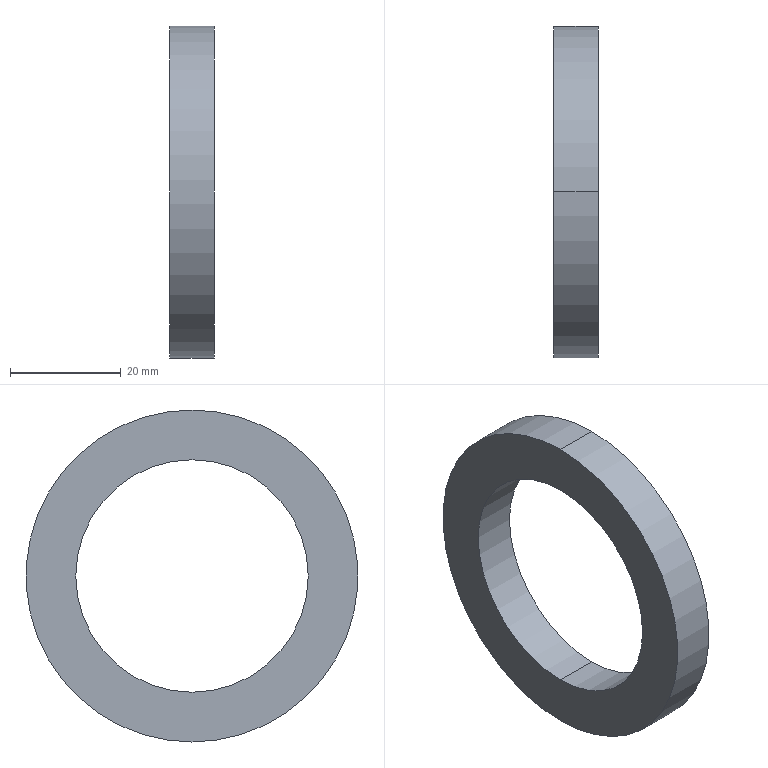Component | SolidWorks | 5ThrustWasher-1 | 1 solid | 6 faces | box 8 x 60 x 60 mm | volume 11536 mm3 | cylinder 4 | plane 2 | commonest cylinder face diameters 42 x2 60 x2
build123d program:
from build123d import *

# Parameters (mm, degrees)
SKETCH1_R           = 30
SKETCH1_R_2         = 21
BOSS_EXTRUDE1_DEPTH = 8


with BuildPart() as part:
    # Sketch1 → Boss-Extrude1 (new body)
    with BuildSketch(Plane(origin=(0, 0, 0), x_dir=(0, 0, -1), z_dir=(1, 0, 0))):
        Circle(SKETCH1_R)
        Circle(SKETCH1_R_2, mode=Mode.SUBTRACT)
    extrude(amount=BOSS_EXTRUDE1_DEPTH)


solid = part.part

# Placed as in the assembly
solid = solid.moved(Location((87.957, 1.776, 250), (0, 0, 0)))
STEP:
#1=COLOUR_RGB('',0.7922,0.8196,0.9333);
#2=FILL_AREA_STYLE_COLOUR('',#1);
#3=FILL_AREA_STYLE('',(#2));
#4=SURFACE_STYLE_FILL_AREA(#3);
#5=SURFACE_SIDE_STYLE('',(#4));
#6=SURFACE_STYLE_USAGE(.BOTH.,#5);
#7=PRESENTATION_STYLE_ASSIGNMENT((#6));
#8=CARTESIAN_POINT('',(3.778,0.06992,10.669));
#9=VERTEX_POINT('',#8);
#10=CARTESIAN_POINT('',(3.778,0.06992,9.016));
#11=VERTEX_POINT('',#10);
#12=CARTESIAN_POINT('',(3.778,0.06992,9.843));
#13=DIRECTION('',(1.,0.,0.));
#14=DIRECTION('',(0.,0.,-1.));
#15=AXIS2_PLACEMENT_3D('',#12,#13,#14);
#16=CIRCLE('',#15,0.8268);
#17=EDGE_CURVE('',#9,#11,#16,.T.);
#18=ORIENTED_EDGE('',*,*,#17,.T.);
#19=CARTESIAN_POINT('',(3.463,0.06992,9.016));
#20=VERTEX_POINT('',#19);
#21=CARTESIAN_POINT('',(3.778,0.06992,9.016));
#22=DIRECTION('',(-1.,0.,0.));
#23=VECTOR('',#22,39.37);
#24=LINE('',#21,#23);
#25=EDGE_CURVE('',#11,#20,#24,.T.);
#26=ORIENTED_EDGE('',*,*,#25,.T.);
#27=CARTESIAN_POINT('',(3.463,0.06992,10.669));
#28=VERTEX_POINT('',#27);
#29=CARTESIAN_POINT('',(3.463,0.06992,9.843));
#30=DIRECTION('',(1.,0.,0.));
#31=DIRECTION('',(0.,0.,-1.));
#32=AXIS2_PLACEMENT_3D('',#29,#30,#31);
#33=CIRCLE('',#32,0.8268);
#34=EDGE_CURVE('',#28,#20,#33,.T.);
#35=ORIENTED_EDGE('',*,*,#34,.F.);
#36=CARTESIAN_POINT('',(3.778,0.06992,10.669));
#37=DIRECTION('',(-1.,0.,0.));
#38=VECTOR('',#37,39.37);
#39=LINE('',#36,#38);
#40=EDGE_CURVE('',#9,#28,#39,.T.);
#41=ORIENTED_EDGE('',*,*,#40,.F.);
#42=EDGE_LOOP('',(#18,#26,#35,#41));
#43=FACE_OUTER_BOUND('',#42,.T.);
#44=CARTESIAN_POINT('',(3.778,0.06992,9.843));
#45=DIRECTION('',(-1.,0.,0.));
#46=DIRECTION('',(0.,0.,1.));
#47=AXIS2_PLACEMENT_3D('',#44,#45,#46);
#48=CYLINDRICAL_SURFACE('',#47,0.8268);
#49=ADVANCED_FACE('',(#43),#48,.F.);
#50=CARTESIAN_POINT('',(3.778,0.06992,8.661));
#51=VERTEX_POINT('',#50);
#52=CARTESIAN_POINT('',(3.778,0.06992,11.024));
#53=VERTEX_POINT('',#52);
#54=CARTESIAN_POINT('',(3.778,0.06992,9.843));
#55=DIRECTION('',(1.,0.,0.));
#56=DIRECTION('',(0.,0.,-1.));
#57=AXIS2_PLACEMENT_3D('',#54,#55,#56);
#58=CIRCLE('',#57,1.181);
#59=EDGE_CURVE('',#51,#53,#58,.T.);
#60=ORIENTED_EDGE('',*,*,#59,.F.);
#61=CARTESIAN_POINT('',(3.463,0.06992,8.661));
#62=VERTEX_POINT('',#61);
#63=CARTESIAN_POINT('',(3.778,0.06992,8.661));
#64=DIRECTION('',(-1.,0.,0.));
#65=VECTOR('',#64,39.37);
#66=LINE('',#63,#65);
#67=EDGE_CURVE('',#51,#62,#66,.T.);
#68=ORIENTED_EDGE('',*,*,#67,.T.);
#69=CARTESIAN_POINT('',(3.463,0.06992,11.024));
#70=VERTEX_POINT('',#69);
#71=CARTESIAN_POINT('',(3.463,0.06992,9.843));
#72=DIRECTION('',(1.,0.,0.));
#73=DIRECTION('',(0.,0.,-1.));
#74=AXIS2_PLACEMENT_3D('',#71,#72,#73);
#75=CIRCLE('',#74,1.181);
#76=EDGE_CURVE('',#62,#70,#75,.T.);
#77=ORIENTED_EDGE('',*,*,#76,.T.);
#78=CARTESIAN_POINT('',(3.778,0.06992,11.024));
#79=DIRECTION('',(-1.,0.,0.));
#80=VECTOR('',#79,39.37);
#81=LINE('',#78,#80);
#82=EDGE_CURVE('',#53,#70,#81,.T.);
#83=ORIENTED_EDGE('',*,*,#82,.F.);
#84=EDGE_LOOP('',(#60,#68,#77,#83));
#85=FACE_OUTER_BOUND('',#84,.T.);
#86=CARTESIAN_POINT('',(3.778,0.06992,9.843));
#87=DIRECTION('',(-1.,0.,0.));
#88=DIRECTION('',(0.,0.,1.));
#89=AXIS2_PLACEMENT_3D('',#86,#87,#88);
#90=CYLINDRICAL_SURFACE('',#89,1.181);
#91=ADVANCED_FACE('',(#85),#90,.T.);
#92=CARTESIAN_POINT('',(3.778,0.06992,9.843));
#93=DIRECTION('',(1.,0.,0.));
#94=DIRECTION('',(0.,0.,-1.));
#95=AXIS2_PLACEMENT_3D('',#92,#93,#94);
#96=CIRCLE('',#95,1.181);
#97=EDGE_CURVE('',#53,#51,#96,.T.);
#98=ORIENTED_EDGE('',*,*,#97,.T.);
#99=ORIENTED_EDGE('',*,*,#59,.T.);
#100=EDGE_LOOP('',(#98,#99));
#101=FACE_OUTER_BOUND('',#100,.T.);
#102=ORIENTED_EDGE('',*,*,#17,.F.);
#103=CARTESIAN_POINT('',(3.778,0.06992,9.843));
#104=DIRECTION('',(1.,0.,0.));
#105=DIRECTION('',(0.,0.,-1.));
#106=AXIS2_PLACEMENT_3D('',#103,#104,#105);
#107=CIRCLE('',#106,0.8268);
#108=EDGE_CURVE('',#11,#9,#107,.T.);
#109=ORIENTED_EDGE('',*,*,#108,.F.);
#110=EDGE_LOOP('',(#102,#109));
#111=FACE_BOUND('',#110,.T.);
#112=CARTESIAN_POINT('',(3.778,0.06992,9.843));
#113=DIRECTION('',(1.,0.,0.));
#114=DIRECTION('',(0.,0.,-1.));
#115=AXIS2_PLACEMENT_3D('',#112,#113,#114);
#116=PLANE('',#115);
#117=ADVANCED_FACE('',(#101,#111),#116,.T.);
#118=CARTESIAN_POINT('',(3.463,0.06992,9.843));
#119=DIRECTION('',(1.,0.,0.));
#120=DIRECTION('',(0.,0.,-1.));
#121=AXIS2_PLACEMENT_3D('',#118,#119,#120);
#122=CIRCLE('',#121,1.181);
#123=EDGE_CURVE('',#70,#62,#122,.T.);
#124=ORIENTED_EDGE('',*,*,#123,.F.);
#125=ORIENTED_EDGE('',*,*,#76,.F.);
#126=EDGE_LOOP('',(#124,#125));
#127=FACE_OUTER_BOUND('',#126,.T.);
#128=ORIENTED_EDGE('',*,*,#34,.T.);
#129=CARTESIAN_POINT('',(3.463,0.06992,9.843));
#130=DIRECTION('',(1.,0.,0.));
#131=DIRECTION('',(0.,0.,-1.));
#132=AXIS2_PLACEMENT_3D('',#129,#130,#131);
#133=CIRCLE('',#132,0.8268);
#134=EDGE_CURVE('',#20,#28,#133,.T.);
#135=ORIENTED_EDGE('',*,*,#134,.T.);
#136=EDGE_LOOP('',(#128,#135));
#137=FACE_BOUND('',#136,.T.);
#138=CARTESIAN_POINT('',(3.463,0.06992,9.843));
#139=DIRECTION('',(1.,0.,0.));
#140=DIRECTION('',(0.,0.,-1.));
#141=AXIS2_PLACEMENT_3D('',#138,#139,#140);
#142=PLANE('',#141);
#143=ADVANCED_FACE('',(#127,#137),#142,.F.);
#144=ORIENTED_EDGE('',*,*,#67,.F.);
#145=ORIENTED_EDGE('',*,*,#97,.F.);
#146=ORIENTED_EDGE('',*,*,#82,.T.);
#147=ORIENTED_EDGE('',*,*,#123,.T.);
#148=EDGE_LOOP('',(#144,#145,#146,#147));
#149=FACE_OUTER_BOUND('',#148,.T.);
#150=CARTESIAN_POINT('',(3.778,0.06992,9.843));
#151=DIRECTION('',(-1.,0.,0.));
#152=DIRECTION('',(0.,0.,1.));
#153=AXIS2_PLACEMENT_3D('',#150,#151,#152);
#154=CYLINDRICAL_SURFACE('',#153,1.181);
#155=ADVANCED_FACE('',(#149),#154,.T.);
#156=ORIENTED_EDGE('',*,*,#25,.F.);
#157=ORIENTED_EDGE('',*,*,#108,.T.);
#158=ORIENTED_EDGE('',*,*,#40,.T.);
#159=ORIENTED_EDGE('',*,*,#134,.F.);
#160=EDGE_LOOP('',(#156,#157,#158,#159));
#161=FACE_OUTER_BOUND('',#160,.T.);
#162=CARTESIAN_POINT('',(3.778,0.06992,9.843));
#163=DIRECTION('',(-1.,0.,0.));
#164=DIRECTION('',(0.,0.,1.));
#165=AXIS2_PLACEMENT_3D('',#162,#163,#164);
#166=CYLINDRICAL_SURFACE('',#165,0.8268);
#167=ADVANCED_FACE('',(#161),#166,.F.);
#168=CLOSED_SHELL('',(#49,#91,#117,#143,#155,#167));
#169=MANIFOLD_SOLID_BREP('',#168);
#170=STYLED_ITEM('',(#7),#169);
#171=(LENGTH_UNIT()NAMED_UNIT(*)SI_UNIT($,.METRE.));
#172=LENGTH_MEASURE_WITH_UNIT(LENGTH_MEASURE(0.0254),#171);
#173=DIMENSIONAL_EXPONENTS(1.,0.,0.,0.,0.,0.,0.);
#174=(CONVERSION_BASED_UNIT('',#172)LENGTH_UNIT()NAMED_UNIT(#173));
#175=UNCERTAINTY_MEASURE_WITH_UNIT(LENGTH_MEASURE(0.00001),#174,'','');
#176=(NAMED_UNIT(*)PLANE_ANGLE_UNIT()SI_UNIT($,.RADIAN.));
#177=(NAMED_UNIT(*)SI_UNIT($,.STERADIAN.)SOLID_ANGLE_UNIT());
#178=(GEOMETRIC_REPRESENTATION_CONTEXT(3)GLOBAL_UNCERTAINTY_ASSIGNED_CONTEXT((#175))GLOBAL_UNIT_ASSIGNED_CONTEXT((#174,#176,#177))REPRESENTATION_CONTEXT('',''));
#179=MECHANICAL_DESIGN_GEOMETRIC_PRESENTATION_REPRESENTATION('',(#170),#178);
#180=PRESENTATION_LAYER_ASSIGNMENT('','',(#170));
#181=CARTESIAN_POINT('',(0.,0.,0.));
#182=DIRECTION('',(0.,0.,1.));
#183=DIRECTION('',(1.,0.,0.));
#184=AXIS2_PLACEMENT_3D('',#181,#182,#183);
#185=(LENGTH_UNIT()NAMED_UNIT(*)SI_UNIT($,.METRE.));
#186=LENGTH_MEASURE_WITH_UNIT(LENGTH_MEASURE(0.0254),#185);
#187=DIMENSIONAL_EXPONENTS(1.,0.,0.,0.,0.,0.,0.);
#188=(CONVERSION_BASED_UNIT('',#186)LENGTH_UNIT()NAMED_UNIT(#187));
#189=UNCERTAINTY_MEASURE_WITH_UNIT(LENGTH_MEASURE(0.00001),#188,'','');
#190=(NAMED_UNIT(*)PLANE_ANGLE_UNIT()SI_UNIT($,.RADIAN.));
#191=(NAMED_UNIT(*)SI_UNIT($,.STERADIAN.)SOLID_ANGLE_UNIT());
#192=(GEOMETRIC_REPRESENTATION_CONTEXT(3)GLOBAL_UNCERTAINTY_ASSIGNED_CONTEXT((#189))GLOBAL_UNIT_ASSIGNED_CONTEXT((#188,#190,#191))REPRESENTATION_CONTEXT('',''));
#193=ADVANCED_BREP_SHAPE_REPRESENTATION('',(#169,#184),#192);